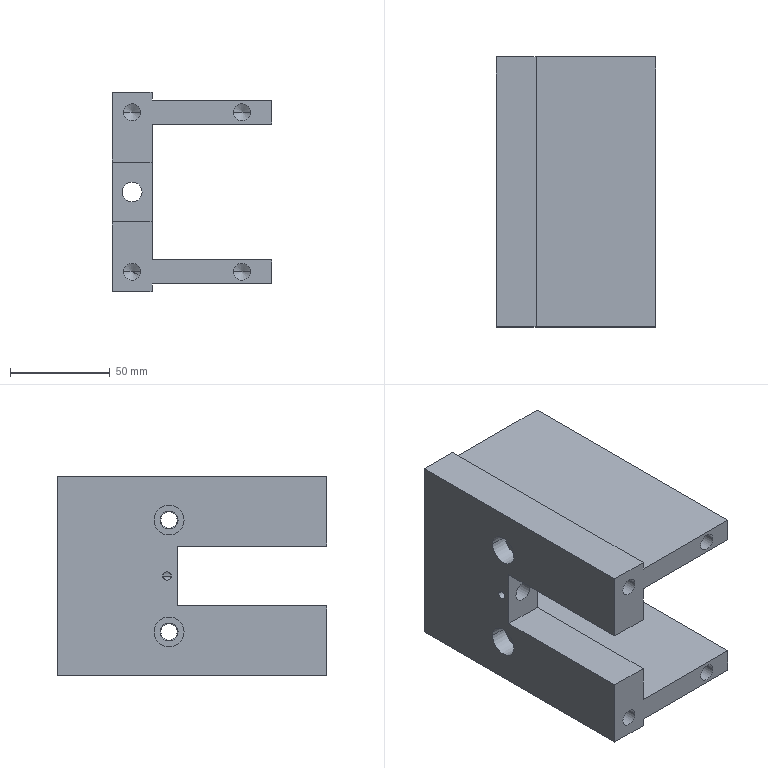Component | SolidWorks | SHYTJ-01-07-03SupportPlate-1 | 1 solid | 71 faces | box 80 x 135 x 100 mm | volume 392405 mm3 | cylinder 30 | plane 21 | cone 20 | commonest cylinder face diameters 8.5 x16 15 x4 9 x4 4.2 x2 16 x2 10 x2
build123d program:
from build123d import *

# Parameters (mm, degrees)
SKETCH1_W                                         = 135
SKETCH1_H                                         = 100
BOSS_EXTRUDE1_DEPTH                               = 20
SKETCH4_W                                         = 135
SKETCH4_H                                         = 12
BOSS_EXTRUDE2_DEPTH                               = 60
M10_TAPPED_HOLE2_D                                = 8.5
M10_TAPPED_HOLE2_DEPTH                            = 24.5
M10_TAPPED_HOLE2_TIP                              = 2.554
M10_TAPPED_HOLE3_D                                = 8.5
M10_TAPPED_HOLE3_DEPTH                            = 24.5
M10_TAPPED_HOLE3_TIP                              = 2.554
SKETCH14_W                                        = 85.192
SKETCH14_H                                        = 30
CUT_EXTRUDE2_DEPTH                                = 30
SKETCH15_R                                        = 5
CUT_EXTRUDE3_DEPTH                                = 139.654
SKETCH16_R                                        = 8
CUT_EXTRUDE4_DEPTH                                = 50
HOLE_SIZE_ACCORDING_TO_TYPE_OF_SOCKET_D           = 9
HOLE_SIZE_ACCORDING_TO_TYPE_OF_SOCKET_DEPTH       = 19.75
HOLE_SIZE_ACCORDING_TO_TYPE_OF_SOCKET_CBORE_D     = 15
HOLE_SIZE_ACCORDING_TO_TYPE_OF_SOCKET_CBORE_DEPTH = 9
HOLE_SIZE_ACCORDING_TO_TYPE_OF_SOCKET_TIP         = 2.704
M5_TAPPED_HOLE1_D                                 = 4.2
M5_TAPPED_HOLE1_DEPTH                             = 12.4
M5_TAPPED_HOLE1_TIP                               = 1.262


with BuildPart() as part:
    # Sketch1 → Boss-Extrude1 (new body)
    with BuildSketch(Plane.XY):
        with Locations((67.5, 50)):
            Rectangle(SKETCH1_W, SKETCH1_H)
    extrude(amount=BOSS_EXTRUDE1_DEPTH)

    # Sketch4 → Boss-Extrude2 (add)
    with BuildSketch(Plane(origin=(0, 0, 0), x_dir=(-1, 0, 0), z_dir=(0, 0, -1))):
        with Locations((-67.5, 90)):
            Rectangle(SKETCH4_W, SKETCH4_H)
        with Locations((-67.5, 10)):
            Rectangle(SKETCH4_W, SKETCH4_H)
    extrude(amount=BOSS_EXTRUDE2_DEPTH)

    # M10 Tapped Hole2
    with Locations(Plane.ZY):
        with Locations((10, 90), (10, 10), (-45, 90), (-45, 10)):
            Hole(M10_TAPPED_HOLE2_D / 2, depth=M10_TAPPED_HOLE2_DEPTH)
            with Locations((0, 0, -(M10_TAPPED_HOLE2_DEPTH + M10_TAPPED_HOLE2_TIP / 2))):  # 118° drill point
                Cone(0, M10_TAPPED_HOLE2_D / 2, M10_TAPPED_HOLE2_TIP, mode=Mode.SUBTRACT)

    # M10 Tapped Hole3
    with Locations(Plane(origin=(135, 0, 0), x_dir=(0, 0, -1), z_dir=(1, 0, 0))):
        with Locations((-9.996, 90), (45.004, 90), (-9.996, 10), (45.004, 10)):
            Hole(M10_TAPPED_HOLE3_D / 2, depth=M10_TAPPED_HOLE3_DEPTH)
            with Locations((0, 0, -(M10_TAPPED_HOLE3_DEPTH + M10_TAPPED_HOLE3_TIP / 2))):  # 118° drill point
                Cone(0, M10_TAPPED_HOLE3_D / 2, M10_TAPPED_HOLE3_TIP, mode=Mode.SUBTRACT)

    # Sketch14 → Cut-Extrude2 (cut)
    with BuildSketch(Plane(origin=(0, 0, 0), x_dir=(-1, 0, 0), z_dir=(0, 0, -1))):
        with Locations((-102.596, 50)):
            Rectangle(SKETCH14_W, SKETCH14_H)
    extrude(amount=-CUT_EXTRUDE2_DEPTH, mode=Mode.SUBTRACT)

    # Sketch15 → Cut-Extrude3 (cut, through all)
    with BuildSketch(Plane(origin=(60, 0, 0), x_dir=(0, 0, -1), z_dir=(1, 0, 0))):
        with Locations((-10, 50)):
            Circle(SKETCH15_R)
    extrude(amount=-CUT_EXTRUDE3_DEPTH, mode=Mode.SUBTRACT)

    # Sketch16 → Cut-Extrude4 (cut)
    with BuildSketch(Plane.ZY):
        with Locations((10, 50)):
            Circle(SKETCH16_R)
    extrude(amount=-CUT_EXTRUDE4_DEPTH, mode=Mode.SUBTRACT)

    # Hole Size _according to_ type of socket
    with Locations(Plane(origin=(0, 0, 20), x_dir=(-1, 0, 0), z_dir=(0, 0, 1))):
        with Locations((-56, -78), (-56, -22)):
            CounterBoreHole(HOLE_SIZE_ACCORDING_TO_TYPE_OF_SOCKET_D / 2, HOLE_SIZE_ACCORDING_TO_TYPE_OF_SOCKET_CBORE_D / 2, HOLE_SIZE_ACCORDING_TO_TYPE_OF_SOCKET_CBORE_DEPTH, depth=HOLE_SIZE_ACCORDING_TO_TYPE_OF_SOCKET_DEPTH)
            with Locations((0, 0, -(HOLE_SIZE_ACCORDING_TO_TYPE_OF_SOCKET_DEPTH + HOLE_SIZE_ACCORDING_TO_TYPE_OF_SOCKET_TIP / 2))):  # 118° drill point
                Cone(0, HOLE_SIZE_ACCORDING_TO_TYPE_OF_SOCKET_D / 2, HOLE_SIZE_ACCORDING_TO_TYPE_OF_SOCKET_TIP, mode=Mode.SUBTRACT)

    # M5 Tapped Hole1
    with Locations(Plane.XY.offset(20)):
        with Locations((55, 50)):
            Hole(M5_TAPPED_HOLE1_D / 2, depth=M5_TAPPED_HOLE1_DEPTH)
            with Locations((0, 0, -(M5_TAPPED_HOLE1_DEPTH + M5_TAPPED_HOLE1_TIP / 2))):  # 118° drill point
                Cone(0, M5_TAPPED_HOLE1_D / 2, M5_TAPPED_HOLE1_TIP, mode=Mode.SUBTRACT)


solid = part.part

# Placed as in the assembly
solid = solid.moved(Location((149.884, -20.361, 220), (90, -90, 0)))